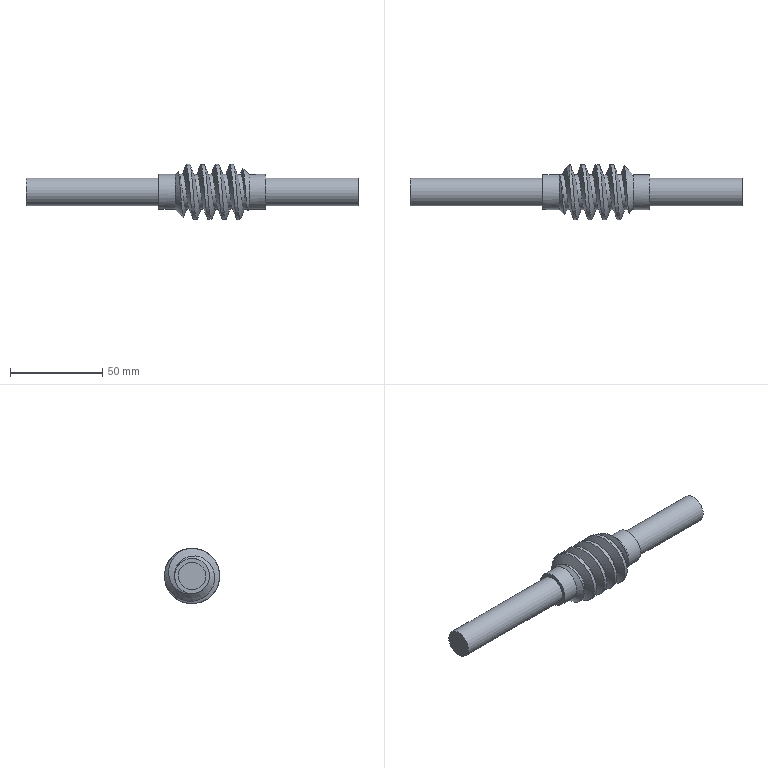Component | NX | WORM | 1 solid | 14 faces | volume 44803 mm3 | cylinder 5 | plane 4 | spline 3 | cone 2 | commonest cylinder face diameters 15 x2 19 x2 30 x1